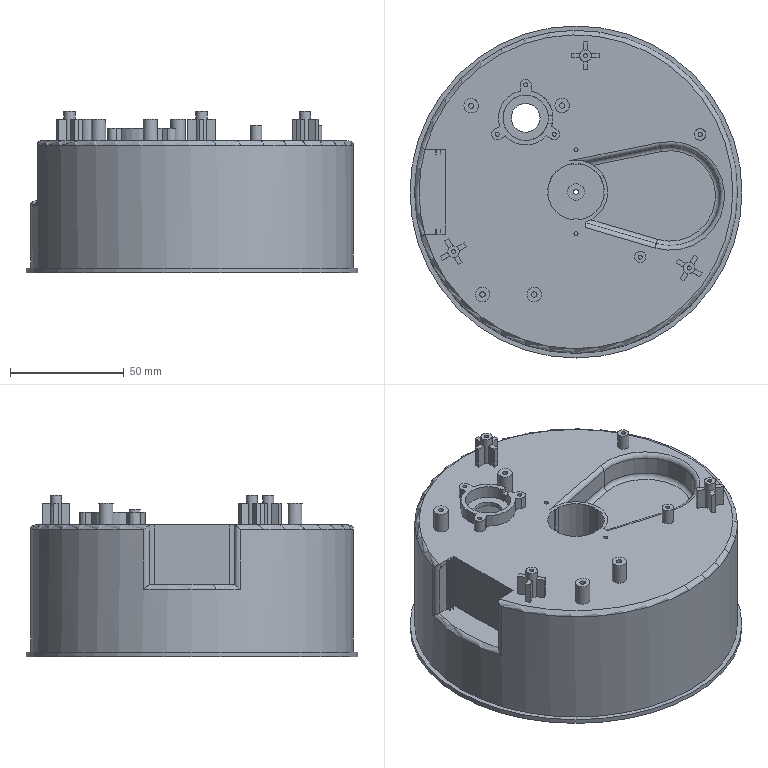Component | NX | INNER_LINER | 1 solid | 255 faces | volume 95786 mm3 | plane 144 | cylinder 79 | torus 18 | spline 7 | sphere 7 | commonest cylinder face diameters 4 x27 1.8 x10 5 x5 23.94 x4 24.9 x4 2.35 x4 6.35 x4 24 x3